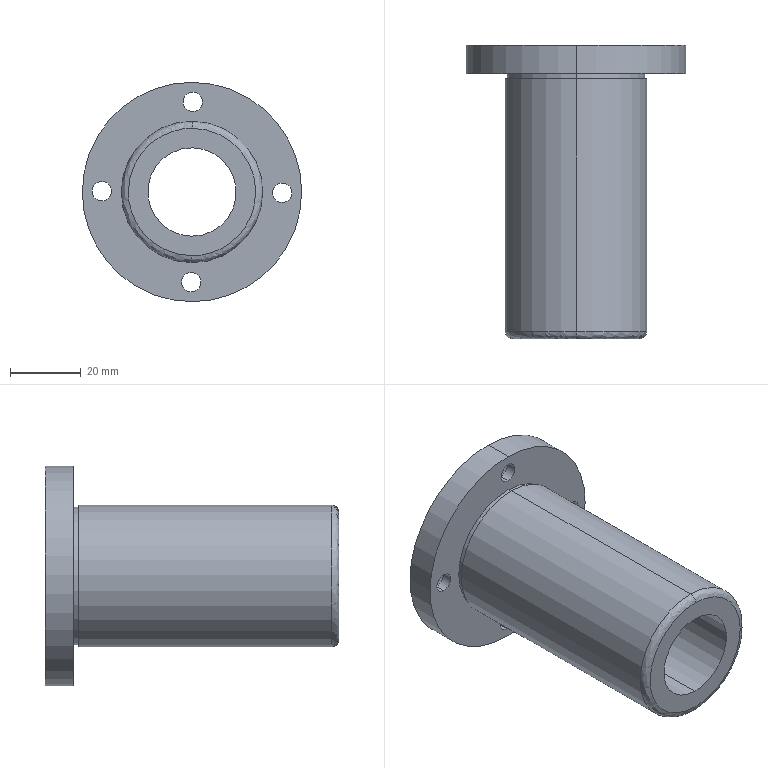Component | SolidWorks | LinearBearingMISUMILHFRD25-1 | 1 solid | 34 faces | box 62 x 83 x 62 mm | volume 75888 mm3 | cylinder 24 | plane 8 | spline 2 | commonest cylinder face diameters 5.5 x8 9 x8 40 x2 39 x2 25 x2 62 x2
STEP:
#1=CARTESIAN_POINT('',(5.125,-0.3937,7.677));
#2=VERTEX_POINT('',#1);
#3=CARTESIAN_POINT('',(5.111,-0.3937,6.102));
#4=VERTEX_POINT('',#3);
#5=CARTESIAN_POINT('',(5.118,-0.3937,6.89));
#6=DIRECTION('',(-0.,1.,-0.));
#7=DIRECTION('',(0.008424,0.,1.));
#8=AXIS2_PLACEMENT_3D('',#5,#6,#7);
#9=CIRCLE('',#8,0.7874);
#10=EDGE_CURVE('',#2,#4,#9,.T.);
#11=ORIENTED_EDGE('',*,*,#10,.F.);
#12=CARTESIAN_POINT('',(5.124,-0.4724,7.598));
#13=VERTEX_POINT('',#12);
#14=CARTESIAN_POINT('',(5.124,-0.3937,7.598));
#15=DIRECTION('',(1.,-0.,-0.008424));
#16=DIRECTION('',(0.008424,0.,1.));
#17=AXIS2_PLACEMENT_3D('',#14,#15,#16);
#18=CIRCLE('',#17,0.07874);
#19=EDGE_CURVE('',#2,#13,#18,.T.);
#20=ORIENTED_EDGE('',*,*,#19,.T.);
#21=CARTESIAN_POINT('',(5.112,-0.4724,6.181));
#22=VERTEX_POINT('',#21);
#23=CARTESIAN_POINT('',(5.124,-0.4724,7.598));
#24=CARTESIAN_POINT('',(6.541,-0.4724,7.586));
#25=CARTESIAN_POINT('',(6.529,-0.4724,6.169));
#26=CARTESIAN_POINT('',(5.112,-0.4724,6.181));
#27=(BOUNDED_CURVE()B_SPLINE_CURVE(3,(#23,#24,#25,#26),.UNSPECIFIED.,.F.,.T.)B_SPLINE_CURVE_WITH_KNOTS((4,4),(0.,1.),.UNSPECIFIED.)CURVE()GEOMETRIC_REPRESENTATION_ITEM()RATIONAL_B_SPLINE_CURVE((1.,0.3333,0.3333,1.))REPRESENTATION_ITEM(''));
#28=EDGE_CURVE('',#13,#22,#27,.T.);
#29=ORIENTED_EDGE('',*,*,#28,.T.);
#30=CARTESIAN_POINT('',(5.112,-0.3937,6.181));
#31=DIRECTION('',(-1.,0.,0.008424));
#32=DIRECTION('',(-0.008424,-0.,-1.));
#33=AXIS2_PLACEMENT_3D('',#30,#31,#32);
#34=CIRCLE('',#33,0.07874);
#35=EDGE_CURVE('',#4,#22,#34,.T.);
#36=ORIENTED_EDGE('',*,*,#35,.F.);
#37=EDGE_LOOP('',(#11,#20,#29,#36));
#38=FACE_OUTER_BOUND('',#37,.T.);
#39=CARTESIAN_POINT('',(5.125,-0.3937,7.677));
#40=CARTESIAN_POINT('',(6.699,-0.3937,7.664));
#41=CARTESIAN_POINT('',(6.686,-0.3937,6.089));
#42=CARTESIAN_POINT('',(5.111,-0.3937,6.102));
#43=CARTESIAN_POINT('',(5.125,-0.4398,7.677));
#44=CARTESIAN_POINT('',(6.699,-0.4398,7.664));
#45=CARTESIAN_POINT('',(6.686,-0.4398,6.089));
#46=CARTESIAN_POINT('',(5.111,-0.4398,6.102));
#47=CARTESIAN_POINT('',(5.124,-0.4724,7.645));
#48=CARTESIAN_POINT('',(6.634,-0.4724,7.632));
#49=CARTESIAN_POINT('',(6.621,-0.4724,6.122));
#50=CARTESIAN_POINT('',(5.112,-0.4724,6.135));
#51=CARTESIAN_POINT('',(5.124,-0.4724,7.598));
#52=CARTESIAN_POINT('',(6.541,-0.4724,7.586));
#53=CARTESIAN_POINT('',(6.529,-0.4724,6.169));
#54=CARTESIAN_POINT('',(5.112,-0.4724,6.181));
#55=(BOUNDED_SURFACE()B_SPLINE_SURFACE(3,3,((#39,#40,#41,#42),(#43,#44,#45,#46),(#47,#48,#49,#50),(#51,#52,#53,#54)),.UNSPECIFIED.,.F.,.F.,.T.)B_SPLINE_SURFACE_WITH_KNOTS((4,4),(4,4),(0.,1.),(0.,1.),.UNSPECIFIED.)GEOMETRIC_REPRESENTATION_ITEM()RATIONAL_B_SPLINE_SURFACE(((1.,0.3333,0.3333,1.),(0.8047,0.2682,0.2682,0.8047),(0.8047,0.2682,0.2682,0.8047),(1.,0.3333,0.3333,1.)))REPRESENTATION_ITEM('')SURFACE());
#56=ADVANCED_FACE('',(#38),#55,.T.);
#57=CARTESIAN_POINT('',(5.125,2.421,7.677));
#58=VERTEX_POINT('',#57);
#59=CARTESIAN_POINT('',(5.111,2.421,6.102));
#60=VERTEX_POINT('',#59);
#61=CARTESIAN_POINT('',(5.118,2.421,6.89));
#62=DIRECTION('',(0.,-1.,0.));
#63=DIRECTION('',(0.008424,0.,1.));
#64=AXIS2_PLACEMENT_3D('',#61,#62,#63);
#65=CIRCLE('',#64,0.7874);
#66=EDGE_CURVE('',#58,#60,#65,.T.);
#67=ORIENTED_EDGE('',*,*,#66,.T.);
#68=CARTESIAN_POINT('',(5.111,1.014,6.102));
#69=DIRECTION('',(0.,-1.,0.));
#70=VECTOR('',#69,39.37);
#71=LINE('',#68,#70);
#72=EDGE_CURVE('',#60,#4,#71,.T.);
#73=ORIENTED_EDGE('',*,*,#72,.T.);
#74=CARTESIAN_POINT('',(5.118,-0.3937,6.89));
#75=DIRECTION('',(-0.,1.,-0.));
#76=DIRECTION('',(0.008424,0.,1.));
#77=AXIS2_PLACEMENT_3D('',#74,#75,#76);
#78=CIRCLE('',#77,0.7874);
#79=EDGE_CURVE('',#4,#2,#78,.T.);
#80=ORIENTED_EDGE('',*,*,#79,.T.);
#81=CARTESIAN_POINT('',(5.125,1.014,7.677));
#82=DIRECTION('',(0.,-1.,0.));
#83=VECTOR('',#82,39.37);
#84=LINE('',#81,#83);
#85=EDGE_CURVE('',#58,#2,#84,.T.);
#86=ORIENTED_EDGE('',*,*,#85,.F.);
#87=EDGE_LOOP('',(#67,#73,#80,#86));
#88=FACE_OUTER_BOUND('',#87,.T.);
#89=CARTESIAN_POINT('',(5.118,1.014,6.89));
#90=DIRECTION('',(0.,-1.,0.));
#91=DIRECTION('',(0.008424,0.,1.));
#92=AXIS2_PLACEMENT_3D('',#89,#90,#91);
#93=CYLINDRICAL_SURFACE('',#92,0.7874);
#94=ADVANCED_FACE('',(#88),#93,.T.);
#95=CARTESIAN_POINT('',(5.125,2.48,7.657));
#96=VERTEX_POINT('',#95);
#97=CARTESIAN_POINT('',(5.112,2.48,6.122));
#98=VERTEX_POINT('',#97);
#99=CARTESIAN_POINT('',(5.118,2.48,6.89));
#100=DIRECTION('',(0.,-1.,0.));
#101=DIRECTION('',(0.008424,0.,1.));
#102=AXIS2_PLACEMENT_3D('',#99,#100,#101);
#103=CIRCLE('',#102,0.7677);
#104=EDGE_CURVE('',#96,#98,#103,.T.);
#105=ORIENTED_EDGE('',*,*,#104,.T.);
#106=CARTESIAN_POINT('',(5.112,2.421,6.122));
#107=VERTEX_POINT('',#106);
#108=CARTESIAN_POINT('',(5.112,2.451,6.122));
#109=DIRECTION('',(0.,-1.,0.));
#110=VECTOR('',#109,39.37);
#111=LINE('',#108,#110);
#112=EDGE_CURVE('',#98,#107,#111,.T.);
#113=ORIENTED_EDGE('',*,*,#112,.T.);
#114=CARTESIAN_POINT('',(5.125,2.421,7.657));
#115=VERTEX_POINT('',#114);
#116=CARTESIAN_POINT('',(5.118,2.421,6.89));
#117=DIRECTION('',(0.,-1.,0.));
#118=DIRECTION('',(0.008424,0.,1.));
#119=AXIS2_PLACEMENT_3D('',#116,#117,#118);
#120=CIRCLE('',#119,0.7677);
#121=EDGE_CURVE('',#115,#107,#120,.T.);
#122=ORIENTED_EDGE('',*,*,#121,.F.);
#123=CARTESIAN_POINT('',(5.125,2.451,7.657));
#124=DIRECTION('',(0.,-1.,0.));
#125=VECTOR('',#124,39.37);
#126=LINE('',#123,#125);
#127=EDGE_CURVE('',#96,#115,#126,.T.);
#128=ORIENTED_EDGE('',*,*,#127,.F.);
#129=EDGE_LOOP('',(#105,#113,#122,#128));
#130=FACE_OUTER_BOUND('',#129,.T.);
#131=CARTESIAN_POINT('',(5.118,2.451,6.89));
#132=DIRECTION('',(0.,-1.,0.));
#133=DIRECTION('',(0.008424,0.,1.));
#134=AXIS2_PLACEMENT_3D('',#131,#132,#133);
#135=CYLINDRICAL_SURFACE('',#134,0.7677);
#136=ADVANCED_FACE('',(#130),#135,.T.);
#137=CARTESIAN_POINT('',(5.114,2.795,6.398));
#138=VERTEX_POINT('',#137);
#139=CARTESIAN_POINT('',(5.122,2.795,7.382));
#140=VERTEX_POINT('',#139);
#141=CARTESIAN_POINT('',(5.118,2.795,6.89));
#142=DIRECTION('',(0.,-1.,0.));
#143=DIRECTION('',(0.008424,0.,1.));
#144=AXIS2_PLACEMENT_3D('',#141,#142,#143);
#145=CIRCLE('',#144,0.4921);
#146=EDGE_CURVE('',#138,#140,#145,.T.);
#147=ORIENTED_EDGE('',*,*,#146,.F.);
#148=CARTESIAN_POINT('',(5.114,-0.4724,6.398));
#149=VERTEX_POINT('',#148);
#150=CARTESIAN_POINT('',(5.114,1.161,6.398));
#151=DIRECTION('',(0.,-1.,0.));
#152=VECTOR('',#151,39.37);
#153=LINE('',#150,#152);
#154=EDGE_CURVE('',#138,#149,#153,.T.);
#155=ORIENTED_EDGE('',*,*,#154,.T.);
#156=CARTESIAN_POINT('',(5.122,-0.4724,7.382));
#157=VERTEX_POINT('',#156);
#158=CARTESIAN_POINT('',(5.118,-0.4724,6.89));
#159=DIRECTION('',(-0.,1.,-0.));
#160=DIRECTION('',(0.008424,0.,1.));
#161=AXIS2_PLACEMENT_3D('',#158,#159,#160);
#162=CIRCLE('',#161,0.4921);
#163=EDGE_CURVE('',#157,#149,#162,.T.);
#164=ORIENTED_EDGE('',*,*,#163,.F.);
#165=CARTESIAN_POINT('',(5.122,1.161,7.382));
#166=DIRECTION('',(0.,-1.,0.));
#167=VECTOR('',#166,39.37);
#168=LINE('',#165,#167);
#169=EDGE_CURVE('',#140,#157,#168,.T.);
#170=ORIENTED_EDGE('',*,*,#169,.F.);
#171=EDGE_LOOP('',(#147,#155,#164,#170));
#172=FACE_OUTER_BOUND('',#171,.T.);
#173=CARTESIAN_POINT('',(5.118,1.161,6.89));
#174=DIRECTION('',(0.,-1.,0.));
#175=DIRECTION('',(0.008424,0.,1.));
#176=AXIS2_PLACEMENT_3D('',#173,#174,#175);
#177=CYLINDRICAL_SURFACE('',#176,0.4921);
#178=ADVANCED_FACE('',(#172),#177,.F.);
#179=CARTESIAN_POINT('',(5.108,2.795,5.669));
#180=VERTEX_POINT('',#179);
#181=CARTESIAN_POINT('',(5.128,2.795,8.11));
#182=VERTEX_POINT('',#181);
#183=CARTESIAN_POINT('',(5.118,2.795,6.89));
#184=DIRECTION('',(-0.,1.,-0.));
#185=DIRECTION('',(0.008424,0.,1.));
#186=AXIS2_PLACEMENT_3D('',#183,#184,#185);
#187=CIRCLE('',#186,1.22);
#188=EDGE_CURVE('',#180,#182,#187,.T.);
#189=ORIENTED_EDGE('',*,*,#188,.F.);
#190=CARTESIAN_POINT('',(5.108,2.48,5.669));
#191=VERTEX_POINT('',#190);
#192=CARTESIAN_POINT('',(5.108,2.638,5.669));
#193=DIRECTION('',(0.,-1.,0.));
#194=VECTOR('',#193,39.37);
#195=LINE('',#192,#194);
#196=EDGE_CURVE('',#180,#191,#195,.T.);
#197=ORIENTED_EDGE('',*,*,#196,.T.);
#198=CARTESIAN_POINT('',(5.128,2.48,8.11));
#199=VERTEX_POINT('',#198);
#200=CARTESIAN_POINT('',(5.118,2.48,6.89));
#201=DIRECTION('',(0.,-1.,0.));
#202=DIRECTION('',(0.008424,0.,1.));
#203=AXIS2_PLACEMENT_3D('',#200,#201,#202);
#204=CIRCLE('',#203,1.22);
#205=EDGE_CURVE('',#199,#191,#204,.T.);
#206=ORIENTED_EDGE('',*,*,#205,.F.);
#207=CARTESIAN_POINT('',(5.128,2.638,8.11));
#208=DIRECTION('',(0.,-1.,0.));
#209=VECTOR('',#208,39.37);
#210=LINE('',#207,#209);
#211=EDGE_CURVE('',#182,#199,#210,.T.);
#212=ORIENTED_EDGE('',*,*,#211,.F.);
#213=EDGE_LOOP('',(#189,#197,#206,#212));
#214=FACE_OUTER_BOUND('',#213,.T.);
#215=CARTESIAN_POINT('',(5.118,2.638,6.89));
#216=DIRECTION('',(0.,-1.,0.));
#217=DIRECTION('',(0.008424,0.,1.));
#218=AXIS2_PLACEMENT_3D('',#215,#216,#217);
#219=CYLINDRICAL_SURFACE('',#218,1.22);
#220=ADVANCED_FACE('',(#214),#219,.T.);
#221=CARTESIAN_POINT('',(4.113,2.594,6.79));
#222=VERTEX_POINT('',#221);
#223=CARTESIAN_POINT('',(4.115,2.594,7.006));
#224=VERTEX_POINT('',#223);
#225=CARTESIAN_POINT('',(4.114,2.594,6.898));
#226=DIRECTION('',(0.,-1.,0.));
#227=DIRECTION('',(0.008424,0.,1.));
#228=AXIS2_PLACEMENT_3D('',#225,#226,#227);
#229=CIRCLE('',#228,0.1083);
#230=EDGE_CURVE('',#222,#224,#229,.T.);
#231=ORIENTED_EDGE('',*,*,#230,.F.);
#232=CARTESIAN_POINT('',(4.113,2.48,6.79));
#233=VERTEX_POINT('',#232);
#234=CARTESIAN_POINT('',(4.113,2.537,6.79));
#235=DIRECTION('',(0.,-1.,0.));
#236=VECTOR('',#235,39.37);
#237=LINE('',#234,#236);
#238=EDGE_CURVE('',#222,#233,#237,.T.);
#239=ORIENTED_EDGE('',*,*,#238,.T.);
#240=CARTESIAN_POINT('',(4.115,2.48,7.006));
#241=VERTEX_POINT('',#240);
#242=CARTESIAN_POINT('',(4.114,2.48,6.898));
#243=DIRECTION('',(-0.,1.,-0.));
#244=DIRECTION('',(0.008424,0.,1.));
#245=AXIS2_PLACEMENT_3D('',#242,#243,#244);
#246=CIRCLE('',#245,0.1083);
#247=EDGE_CURVE('',#241,#233,#246,.T.);
#248=ORIENTED_EDGE('',*,*,#247,.F.);
#249=CARTESIAN_POINT('',(4.115,2.537,7.006));
#250=DIRECTION('',(0.,-1.,0.));
#251=VECTOR('',#250,39.37);
#252=LINE('',#249,#251);
#253=EDGE_CURVE('',#224,#241,#252,.T.);
#254=ORIENTED_EDGE('',*,*,#253,.F.);
#255=EDGE_LOOP('',(#231,#239,#248,#254));
#256=FACE_OUTER_BOUND('',#255,.T.);
#257=CARTESIAN_POINT('',(4.114,2.537,6.898));
#258=DIRECTION('',(0.,-1.,0.));
#259=DIRECTION('',(0.008424,0.,1.));
#260=AXIS2_PLACEMENT_3D('',#257,#258,#259);
#261=CYLINDRICAL_SURFACE('',#260,0.1083);
#262=ADVANCED_FACE('',(#256),#261,.F.);
#263=CARTESIAN_POINT('',(5.126,2.594,7.785));
#264=VERTEX_POINT('',#263);
#265=CARTESIAN_POINT('',(5.127,2.594,8.002));
#266=VERTEX_POINT('',#265);
#267=CARTESIAN_POINT('',(5.127,2.594,7.894));
#268=DIRECTION('',(0.,-1.,0.));
#269=DIRECTION('',(0.008424,0.,1.));
#270=AXIS2_PLACEMENT_3D('',#267,#268,#269);
#271=CIRCLE('',#270,0.1083);
#272=EDGE_CURVE('',#264,#266,#271,.T.);
#273=ORIENTED_EDGE('',*,*,#272,.F.);
#274=CARTESIAN_POINT('',(5.126,2.48,7.785));
#275=VERTEX_POINT('',#274);
#276=CARTESIAN_POINT('',(5.126,2.537,7.785));
#277=DIRECTION('',(0.,-1.,0.));
#278=VECTOR('',#277,39.37);
#279=LINE('',#276,#278);
#280=EDGE_CURVE('',#264,#275,#279,.T.);
#281=ORIENTED_EDGE('',*,*,#280,.T.);
#282=CARTESIAN_POINT('',(5.127,2.48,8.002));
#283=VERTEX_POINT('',#282);
#284=CARTESIAN_POINT('',(5.127,2.48,7.894));
#285=DIRECTION('',(-0.,1.,-0.));
#286=DIRECTION('',(0.008424,0.,1.));
#287=AXIS2_PLACEMENT_3D('',#284,#285,#286);
#288=CIRCLE('',#287,0.1083);
#289=EDGE_CURVE('',#283,#275,#288,.T.);
#290=ORIENTED_EDGE('',*,*,#289,.F.);
#291=CARTESIAN_POINT('',(5.127,2.537,8.002));
#292=DIRECTION('',(0.,-1.,0.));
#293=VECTOR('',#292,39.37);
#294=LINE('',#291,#293);
#295=EDGE_CURVE('',#266,#283,#294,.T.);
#296=ORIENTED_EDGE('',*,*,#295,.F.);
#297=EDGE_LOOP('',(#273,#281,#290,#296));
#298=FACE_OUTER_BOUND('',#297,.T.);
#299=CARTESIAN_POINT('',(5.127,2.537,7.894));
#300=DIRECTION('',(0.,-1.,0.));
#301=DIRECTION('',(0.008424,0.,1.));
#302=AXIS2_PLACEMENT_3D('',#299,#300,#301);
#303=CYLINDRICAL_SURFACE('',#302,0.1083);
#304=ADVANCED_FACE('',(#298),#303,.F.);
#305=CARTESIAN_POINT('',(6.121,2.594,6.773));
#306=VERTEX_POINT('',#305);
#307=CARTESIAN_POINT('',(6.123,2.594,6.99));
#308=VERTEX_POINT('',#307);
#309=CARTESIAN_POINT('',(6.122,2.594,6.881));
#310=DIRECTION('',(0.,-1.,0.));
#311=DIRECTION('',(0.008424,0.,1.));
#312=AXIS2_PLACEMENT_3D('',#309,#310,#311);
#313=CIRCLE('',#312,0.1083);
#314=EDGE_CURVE('',#306,#308,#313,.T.);
#315=ORIENTED_EDGE('',*,*,#314,.F.);
#316=CARTESIAN_POINT('',(6.121,2.48,6.773));
#317=VERTEX_POINT('',#316);
#318=CARTESIAN_POINT('',(6.121,2.537,6.773));
#319=DIRECTION('',(0.,-1.,0.));
#320=VECTOR('',#319,39.37);
#321=LINE('',#318,#320);
#322=EDGE_CURVE('',#306,#317,#321,.T.);
#323=ORIENTED_EDGE('',*,*,#322,.T.);
#324=CARTESIAN_POINT('',(6.123,2.48,6.99));
#325=VERTEX_POINT('',#324);
#326=CARTESIAN_POINT('',(6.122,2.48,6.881));
#327=DIRECTION('',(-0.,1.,-0.));
#328=DIRECTION('',(0.008424,0.,1.));
#329=AXIS2_PLACEMENT_3D('',#326,#327,#328);
#330=CIRCLE('',#329,0.1083);
#331=EDGE_CURVE('',#325,#317,#330,.T.);
#332=ORIENTED_EDGE('',*,*,#331,.F.);
#333=CARTESIAN_POINT('',(6.123,2.537,6.99));
#334=DIRECTION('',(0.,-1.,0.));
#335=VECTOR('',#334,39.37);
#336=LINE('',#333,#335);
#337=EDGE_CURVE('',#308,#325,#336,.T.);
#338=ORIENTED_EDGE('',*,*,#337,.F.);
#339=EDGE_LOOP('',(#315,#323,#332,#338));
#340=FACE_OUTER_BOUND('',#339,.T.);
#341=CARTESIAN_POINT('',(6.122,2.537,6.881));
#342=DIRECTION('',(0.,-1.,0.));
#343=DIRECTION('',(0.008424,0.,1.));
#344=AXIS2_PLACEMENT_3D('',#341,#342,#343);
#345=CYLINDRICAL_SURFACE('',#344,0.1083);
#346=ADVANCED_FACE('',(#340),#345,.F.);
#347=CARTESIAN_POINT('',(5.109,2.594,5.778));
#348=VERTEX_POINT('',#347);
#349=CARTESIAN_POINT('',(5.111,2.594,5.994));
#350=VERTEX_POINT('',#349);
#351=CARTESIAN_POINT('',(5.11,2.594,5.886));
#352=DIRECTION('',(0.,-1.,0.));
#353=DIRECTION('',(0.008424,0.,1.));
#354=AXIS2_PLACEMENT_3D('',#351,#352,#353);
#355=CIRCLE('',#354,0.1083);
#356=EDGE_CURVE('',#348,#350,#355,.T.);
#357=ORIENTED_EDGE('',*,*,#356,.F.);
#358=CARTESIAN_POINT('',(5.109,2.48,5.778));
#359=VERTEX_POINT('',#358);
#360=CARTESIAN_POINT('',(5.109,2.537,5.778));
#361=DIRECTION('',(0.,-1.,0.));
#362=VECTOR('',#361,39.37);
#363=LINE('',#360,#362);
#364=EDGE_CURVE('',#348,#359,#363,.T.);
#365=ORIENTED_EDGE('',*,*,#364,.T.);
#366=CARTESIAN_POINT('',(5.111,2.48,5.994));
#367=VERTEX_POINT('',#366);
#368=CARTESIAN_POINT('',(5.11,2.48,5.886));
#369=DIRECTION('',(-0.,1.,-0.));
#370=DIRECTION('',(0.008424,0.,1.));
#371=AXIS2_PLACEMENT_3D('',#368,#369,#370);
#372=CIRCLE('',#371,0.1083);
#373=EDGE_CURVE('',#367,#359,#372,.T.);
#374=ORIENTED_EDGE('',*,*,#373,.F.);
#375=CARTESIAN_POINT('',(5.111,2.537,5.994));
#376=DIRECTION('',(0.,-1.,0.));
#377=VECTOR('',#376,39.37);
#378=LINE('',#375,#377);
#379=EDGE_CURVE('',#350,#367,#378,.T.);
#380=ORIENTED_EDGE('',*,*,#379,.F.);
#381=EDGE_LOOP('',(#357,#365,#374,#380));
#382=FACE_OUTER_BOUND('',#381,.T.);
#383=CARTESIAN_POINT('',(5.11,2.537,5.886));
#384=DIRECTION('',(0.,-1.,0.));
#385=DIRECTION('',(0.008424,0.,1.));
#386=AXIS2_PLACEMENT_3D('',#383,#384,#385);
#387=CYLINDRICAL_SURFACE('',#386,0.1083);
#388=ADVANCED_FACE('',(#382),#387,.F.);
#389=CARTESIAN_POINT('',(4.113,2.795,6.721));
#390=VERTEX_POINT('',#389);
#391=CARTESIAN_POINT('',(4.116,2.795,7.075));
#392=VERTEX_POINT('',#391);
#393=CARTESIAN_POINT('',(4.114,2.795,6.898));
#394=DIRECTION('',(0.,-1.,0.));
#395=DIRECTION('',(0.008424,0.,1.));
#396=AXIS2_PLACEMENT_3D('',#393,#394,#395);
#397=CIRCLE('',#396,0.1772);
#398=EDGE_CURVE('',#390,#392,#397,.T.);
#399=ORIENTED_EDGE('',*,*,#398,.F.);
#400=CARTESIAN_POINT('',(4.113,2.594,6.721));
#401=VERTEX_POINT('',#400);
#402=CARTESIAN_POINT('',(4.113,2.695,6.721));
#403=DIRECTION('',(0.,-1.,0.));
#404=VECTOR('',#403,39.37);
#405=LINE('',#402,#404);
#406=EDGE_CURVE('',#390,#401,#405,.T.);
#407=ORIENTED_EDGE('',*,*,#406,.T.);
#408=CARTESIAN_POINT('',(4.116,2.594,7.075));
#409=VERTEX_POINT('',#408);
#410=CARTESIAN_POINT('',(4.114,2.594,6.898));
#411=DIRECTION('',(-0.,1.,-0.));
#412=DIRECTION('',(0.008424,0.,1.));
#413=AXIS2_PLACEMENT_3D('',#410,#411,#412);
#414=CIRCLE('',#413,0.1772);
#415=EDGE_CURVE('',#409,#401,#414,.T.);
#416=ORIENTED_EDGE('',*,*,#415,.F.);
#417=CARTESIAN_POINT('',(4.116,2.695,7.075));
#418=DIRECTION('',(0.,-1.,0.));
#419=VECTOR('',#418,39.37);
#420=LINE('',#417,#419);
#421=EDGE_CURVE('',#392,#409,#420,.T.);
#422=ORIENTED_EDGE('',*,*,#421,.F.);
#423=EDGE_LOOP('',(#399,#407,#416,#422));
#424=FACE_OUTER_BOUND('',#423,.T.);
#425=CARTESIAN_POINT('',(4.114,2.695,6.898));
#426=DIRECTION('',(0.,-1.,0.));
#427=DIRECTION('',(0.008424,0.,1.));
#428=AXIS2_PLACEMENT_3D('',#425,#426,#427);
#429=CYLINDRICAL_SURFACE('',#428,0.1772);
#430=ADVANCED_FACE('',(#424),#429,.F.);
#431=CARTESIAN_POINT('',(5.125,2.795,7.717));
#432=VERTEX_POINT('',#431);
#433=CARTESIAN_POINT('',(5.128,2.795,8.071));
#434=VERTEX_POINT('',#433);
#435=CARTESIAN_POINT('',(5.127,2.795,7.894));
#436=DIRECTION('',(0.,-1.,0.));
#437=DIRECTION('',(0.008424,0.,1.));
#438=AXIS2_PLACEMENT_3D('',#435,#436,#437);
#439=CIRCLE('',#438,0.1772);
#440=EDGE_CURVE('',#432,#434,#439,.T.);
#441=ORIENTED_EDGE('',*,*,#440,.F.);
#442=CARTESIAN_POINT('',(5.125,2.594,7.717));
#443=VERTEX_POINT('',#442);
#444=CARTESIAN_POINT('',(5.125,2.695,7.717));
#445=DIRECTION('',(0.,-1.,0.));
#446=VECTOR('',#445,39.37);
#447=LINE('',#444,#446);
#448=EDGE_CURVE('',#432,#443,#447,.T.);
#449=ORIENTED_EDGE('',*,*,#448,.T.);
#450=CARTESIAN_POINT('',(5.128,2.594,8.071));
#451=VERTEX_POINT('',#450);
#452=CARTESIAN_POINT('',(5.127,2.594,7.894));
#453=DIRECTION('',(-0.,1.,-0.));
#454=DIRECTION('',(0.008424,0.,1.));
#455=AXIS2_PLACEMENT_3D('',#452,#453,#454);
#456=CIRCLE('',#455,0.1772);
#457=EDGE_CURVE('',#451,#443,#456,.T.);
#458=ORIENTED_EDGE('',*,*,#457,.F.);
#459=CARTESIAN_POINT('',(5.128,2.695,8.071));
#460=DIRECTION('',(0.,-1.,0.));
#461=VECTOR('',#460,39.37);
#462=LINE('',#459,#461);
#463=EDGE_CURVE('',#434,#451,#462,.T.);
#464=ORIENTED_EDGE('',*,*,#463,.F.);
#465=EDGE_LOOP('',(#441,#449,#458,#464));
#466=FACE_OUTER_BOUND('',#465,.T.);
#467=CARTESIAN_POINT('',(5.127,2.695,7.894));
#468=DIRECTION('',(0.,-1.,0.));
#469=DIRECTION('',(0.008424,0.,1.));
#470=AXIS2_PLACEMENT_3D('',#467,#468,#469);
#471=CYLINDRICAL_SURFACE('',#470,0.1772);
#472=ADVANCED_FACE('',(#466),#471,.F.);
#473=CARTESIAN_POINT('',(6.121,2.795,6.704));
#474=VERTEX_POINT('',#473);
#475=CARTESIAN_POINT('',(6.124,2.795,7.058));
#476=VERTEX_POINT('',#475);
#477=CARTESIAN_POINT('',(6.122,2.795,6.881));
#478=DIRECTION('',(0.,-1.,0.));
#479=DIRECTION('',(0.008424,0.,1.));
#480=AXIS2_PLACEMENT_3D('',#477,#478,#479);
#481=CIRCLE('',#480,0.1772);
#482=EDGE_CURVE('',#474,#476,#481,.T.);
#483=ORIENTED_EDGE('',*,*,#482,.F.);
#484=CARTESIAN_POINT('',(6.121,2.594,6.704));
#485=VERTEX_POINT('',#484);
#486=CARTESIAN_POINT('',(6.121,2.695,6.704));
#487=DIRECTION('',(0.,-1.,0.));
#488=VECTOR('',#487,39.37);
#489=LINE('',#486,#488);
#490=EDGE_CURVE('',#474,#485,#489,.T.);
#491=ORIENTED_EDGE('',*,*,#490,.T.);
#492=CARTESIAN_POINT('',(6.124,2.594,7.058));
#493=VERTEX_POINT('',#492);
#494=CARTESIAN_POINT('',(6.122,2.594,6.881));
#495=DIRECTION('',(-0.,1.,-0.));
#496=DIRECTION('',(0.008424,0.,1.));
#497=AXIS2_PLACEMENT_3D('',#494,#495,#496);
#498=CIRCLE('',#497,0.1772);
#499=EDGE_CURVE('',#493,#485,#498,.T.);
#500=ORIENTED_EDGE('',*,*,#499,.F.);
#501=CARTESIAN_POINT('',(6.124,2.695,7.058));
#502=DIRECTION('',(0.,-1.,0.));
#503=VECTOR('',#502,39.37);
#504=LINE('',#501,#503);
#505=EDGE_CURVE('',#476,#493,#504,.T.);
#506=ORIENTED_EDGE('',*,*,#505,.F.);
#507=EDGE_LOOP('',(#483,#491,#500,#506));
#508=FACE_OUTER_BOUND('',#507,.T.);
#509=CARTESIAN_POINT('',(6.122,2.695,6.881));
#510=DIRECTION('',(0.,-1.,0.));
#511=DIRECTION('',(0.008424,0.,1.));
#512=AXIS2_PLACEMENT_3D('',#509,#510,#511);
#513=CYLINDRICAL_SURFACE('',#512,0.1772);
#514=ADVANCED_FACE('',(#508),#513,.F.);
#515=CARTESIAN_POINT('',(5.108,2.795,5.709));
#516=VERTEX_POINT('',#515);
#517=CARTESIAN_POINT('',(5.111,2.795,6.063));
#518=VERTEX_POINT('',#517);
#519=CARTESIAN_POINT('',(5.11,2.795,5.886));
#520=DIRECTION('',(0.,-1.,0.));
#521=DIRECTION('',(0.008424,0.,1.));
#522=AXIS2_PLACEMENT_3D('',#519,#520,#521);
#523=CIRCLE('',#522,0.1772);
#524=EDGE_CURVE('',#516,#518,#523,.T.);
#525=ORIENTED_EDGE('',*,*,#524,.F.);
#526=CARTESIAN_POINT('',(5.108,2.594,5.709));
#527=VERTEX_POINT('',#526);
#528=CARTESIAN_POINT('',(5.108,2.695,5.709));
#529=DIRECTION('',(0.,-1.,0.));
#530=VECTOR('',#529,39.37);
#531=LINE('',#528,#530);
#532=EDGE_CURVE('',#516,#527,#531,.T.);
#533=ORIENTED_EDGE('',*,*,#532,.T.);
#534=CARTESIAN_POINT('',(5.111,2.594,6.063));
#535=VERTEX_POINT('',#534);
#536=CARTESIAN_POINT('',(5.11,2.594,5.886));
#537=DIRECTION('',(-0.,1.,-0.));
#538=DIRECTION('',(0.008424,0.,1.));
#539=AXIS2_PLACEMENT_3D('',#536,#537,#538);
#540=CIRCLE('',#539,0.1772);
#541=EDGE_CURVE('',#535,#527,#540,.T.);
#542=ORIENTED_EDGE('',*,*,#541,.F.);
#543=CARTESIAN_POINT('',(5.111,2.695,6.063));
#544=DIRECTION('',(0.,-1.,0.));
#545=VECTOR('',#544,39.37);
#546=LINE('',#543,#545);
#547=EDGE_CURVE('',#518,#535,#546,.T.);
#548=ORIENTED_EDGE('',*,*,#547,.F.);
#549=EDGE_LOOP('',(#525,#533,#542,#548));
#550=FACE_OUTER_BOUND('',#549,.T.);
#551=CARTESIAN_POINT('',(5.11,2.695,5.886));
#552=DIRECTION('',(0.,-1.,0.));
#553=DIRECTION('',(0.008424,0.,1.));
#554=AXIS2_PLACEMENT_3D('',#551,#552,#553);
#555=CYLINDRICAL_SURFACE('',#554,0.1772);
#556=ADVANCED_FACE('',(#550),#555,.F.);
#557=ORIENTED_EDGE('',*,*,#72,.F.);
#558=CARTESIAN_POINT('',(5.118,2.421,6.89));
#559=DIRECTION('',(0.,-1.,0.));
#560=DIRECTION('',(0.008424,0.,1.));
#561=AXIS2_PLACEMENT_3D('',#558,#559,#560);
#562=CIRCLE('',#561,0.7874);
#563=EDGE_CURVE('',#60,#58,#562,.T.);
#564=ORIENTED_EDGE('',*,*,#563,.T.);
#565=ORIENTED_EDGE('',*,*,#85,.T.);
#566=ORIENTED_EDGE('',*,*,#10,.T.);
#567=EDGE_LOOP('',(#557,#564,#565,#566));
#568=FACE_OUTER_BOUND('',#567,.T.);
#569=CARTESIAN_POINT('',(5.118,1.014,6.89));
#570=DIRECTION('',(0.,-1.,0.));
#571=DIRECTION('',(0.008424,0.,1.));
#572=AXIS2_PLACEMENT_3D('',#569,#570,#571);
#573=CYLINDRICAL_SURFACE('',#572,0.7874);
#574=ADVANCED_FACE('',(#568),#573,.T.);
#575=ORIENTED_EDGE('',*,*,#19,.F.);
#576=ORIENTED_EDGE('',*,*,#79,.F.);
#577=ORIENTED_EDGE('',*,*,#35,.T.);
#578=CARTESIAN_POINT('',(4.409,-0.4724,6.896));
#579=VERTEX_POINT('',#578);
#580=CARTESIAN_POINT('',(5.112,-0.4724,6.181));
#581=CARTESIAN_POINT('',(4.697,-0.4724,6.185));
#582=CARTESIAN_POINT('',(4.406,-0.4724,6.481));
#583=CARTESIAN_POINT('',(4.409,-0.4724,6.896));
#584=(BOUNDED_CURVE()B_SPLINE_CURVE(3,(#580,#581,#582,#583),.UNSPECIFIED.,.F.,.T.)B_SPLINE_CURVE_WITH_KNOTS((4,4),(0.,1.),.UNSPECIFIED.)CURVE()GEOMETRIC_REPRESENTATION_ITEM()RATIONAL_B_SPLINE_CURVE((1.,0.8047,0.8047,1.))REPRESENTATION_ITEM(''));
#585=EDGE_CURVE('',#22,#579,#584,.T.);
#586=ORIENTED_EDGE('',*,*,#585,.T.);
#587=CARTESIAN_POINT('',(4.409,-0.4724,6.896));
#588=CARTESIAN_POINT('',(4.413,-0.4724,7.311));
#589=CARTESIAN_POINT('',(4.709,-0.4724,7.602));
#590=CARTESIAN_POINT('',(5.124,-0.4724,7.598));
#591=(BOUNDED_CURVE()B_SPLINE_CURVE(3,(#587,#588,#589,#590),.UNSPECIFIED.,.F.,.T.)B_SPLINE_CURVE_WITH_KNOTS((4,4),(0.,1.),.UNSPECIFIED.)CURVE()GEOMETRIC_REPRESENTATION_ITEM()RATIONAL_B_SPLINE_CURVE((1.,0.8047,0.8047,1.))REPRESENTATION_ITEM(''));
#592=EDGE_CURVE('',#579,#13,#591,.T.);
#593=ORIENTED_EDGE('',*,*,#592,.T.);
#594=EDGE_LOOP('',(#575,#576,#577,#586,#593));
#595=FACE_OUTER_BOUND('',#594,.T.);
#596=CARTESIAN_POINT('',(5.111,-0.3937,6.102));
#597=CARTESIAN_POINT('',(3.537,-0.3937,6.116));
#598=CARTESIAN_POINT('',(3.55,-0.3937,7.69));
#599=CARTESIAN_POINT('',(5.125,-0.3937,7.677));
#600=CARTESIAN_POINT('',(5.111,-0.4398,6.102));
#601=CARTESIAN_POINT('',(3.537,-0.4398,6.116));
#602=CARTESIAN_POINT('',(3.55,-0.4398,7.69));
#603=CARTESIAN_POINT('',(5.125,-0.4398,7.677));
#604=CARTESIAN_POINT('',(5.112,-0.4724,6.135));
#605=CARTESIAN_POINT('',(3.602,-0.4724,6.148));
#606=CARTESIAN_POINT('',(3.615,-0.4724,7.657));
#607=CARTESIAN_POINT('',(5.124,-0.4724,7.645));
#608=CARTESIAN_POINT('',(5.112,-0.4724,6.181));
#609=CARTESIAN_POINT('',(3.695,-0.4724,6.193));
#610=CARTESIAN_POINT('',(3.707,-0.4724,7.61));
#611=CARTESIAN_POINT('',(5.124,-0.4724,7.598));
#612=(BOUNDED_SURFACE()B_SPLINE_SURFACE(3,3,((#596,#597,#598,#599),(#600,#601,#602,#603),(#604,#605,#606,#607),(#608,#609,#610,#611)),.UNSPECIFIED.,.F.,.F.,.T.)B_SPLINE_SURFACE_WITH_KNOTS((4,4),(4,4),(0.,1.),(0.,1.),.UNSPECIFIED.)GEOMETRIC_REPRESENTATION_ITEM()RATIONAL_B_SPLINE_SURFACE(((1.,0.3333,0.3333,1.),(0.8047,0.2682,0.2682,0.8047),(0.8047,0.2682,0.2682,0.8047),(1.,0.3333,0.3333,1.)))REPRESENTATION_ITEM('')SURFACE());
#613=ADVANCED_FACE('',(#595),#612,.T.);
#614=ORIENTED_EDGE('',*,*,#66,.F.);
#615=ORIENTED_EDGE('',*,*,#563,.F.);
#616=EDGE_LOOP('',(#614,#615));
#617=FACE_OUTER_BOUND('',#616,.T.);
#618=ORIENTED_EDGE('',*,*,#121,.T.);
#619=CARTESIAN_POINT('',(5.118,2.421,6.89));
#620=DIRECTION('',(0.,-1.,0.));
#621=DIRECTION('',(0.008424,0.,1.));
#622=AXIS2_PLACEMENT_3D('',#619,#620,#621);
#623=CIRCLE('',#622,0.7677);
#624=EDGE_CURVE('',#107,#115,#623,.T.);
#625=ORIENTED_EDGE('',*,*,#624,.T.);
#626=EDGE_LOOP('',(#618,#625));
#627=FACE_BOUND('',#626,.T.);
#628=CARTESIAN_POINT('',(4.341,2.421,6.896));
#629=DIRECTION('',(-0.,1.,-0.));
#630=DIRECTION('',(-0.008424,-0.,-1.));
#631=AXIS2_PLACEMENT_3D('',#628,#629,#630);
#632=PLANE('',#631);
#633=ADVANCED_FACE('',(#617,#627),#632,.T.);
#634=ORIENTED_EDGE('',*,*,#163,.T.);
#635=CARTESIAN_POINT('',(5.118,-0.4724,6.89));
#636=DIRECTION('',(-0.,1.,-0.));
#637=DIRECTION('',(0.008424,0.,1.));
#638=AXIS2_PLACEMENT_3D('',#635,#636,#637);
#639=CIRCLE('',#638,0.4921);
#640=EDGE_CURVE('',#149,#157,#639,.T.);
#641=ORIENTED_EDGE('',*,*,#640,.T.);
#642=EDGE_LOOP('',(#634,#641));
#643=FACE_BOUND('',#642,.T.);
#644=ORIENTED_EDGE('',*,*,#585,.F.);
#645=ORIENTED_EDGE('',*,*,#28,.F.);
#646=ORIENTED_EDGE('',*,*,#592,.F.);
#647=EDGE_LOOP('',(#644,#645,#646));
#648=FACE_OUTER_BOUND('',#647,.T.);
#649=CARTESIAN_POINT('',(4.518,-0.4724,6.895));
#650=DIRECTION('',(0.,-1.,0.));
#651=DIRECTION('',(0.008424,0.,1.));
#652=AXIS2_PLACEMENT_3D('',#649,#650,#651);
#653=PLANE('',#652);
#654=ADVANCED_FACE('',(#643,#648),#653,.T.);
#655=ORIENTED_EDGE('',*,*,#112,.F.);
#656=CARTESIAN_POINT('',(5.118,2.48,6.89));
#657=DIRECTION('',(0.,-1.,0.));
#658=DIRECTION('',(0.008424,0.,1.));
#659=AXIS2_PLACEMENT_3D('',#656,#657,#658);
#660=CIRCLE('',#659,0.7677);
#661=EDGE_CURVE('',#98,#96,#660,.T.);
#662=ORIENTED_EDGE('',*,*,#661,.T.);
#663=ORIENTED_EDGE('',*,*,#127,.T.);
#664=ORIENTED_EDGE('',*,*,#624,.F.);
#665=EDGE_LOOP('',(#655,#662,#663,#664));
#666=FACE_OUTER_BOUND('',#665,.T.);
#667=CARTESIAN_POINT('',(5.118,2.451,6.89));
#668=DIRECTION('',(0.,-1.,0.));
#669=DIRECTION('',(0.008424,0.,1.));
#670=AXIS2_PLACEMENT_3D('',#667,#668,#669);
#671=CYLINDRICAL_SURFACE('',#670,0.7677);
#672=ADVANCED_FACE('',(#666),#671,.T.);
#673=ORIENTED_EDGE('',*,*,#154,.F.);
#674=CARTESIAN_POINT('',(5.118,2.795,6.89));
#675=DIRECTION('',(0.,-1.,0.));
#676=DIRECTION('',(0.008424,0.,1.));
#677=AXIS2_PLACEMENT_3D('',#674,#675,#676);
#678=CIRCLE('',#677,0.4921);
#679=EDGE_CURVE('',#140,#138,#678,.T.);
#680=ORIENTED_EDGE('',*,*,#679,.F.);
#681=ORIENTED_EDGE('',*,*,#169,.T.);
#682=ORIENTED_EDGE('',*,*,#640,.F.);
#683=EDGE_LOOP('',(#673,#680,#681,#682));
#684=FACE_OUTER_BOUND('',#683,.T.);
#685=CARTESIAN_POINT('',(5.118,1.161,6.89));
#686=DIRECTION('',(0.,-1.,0.));
#687=DIRECTION('',(0.008424,0.,1.));
#688=AXIS2_PLACEMENT_3D('',#685,#686,#687);
#689=CYLINDRICAL_SURFACE('',#688,0.4921);
#690=ADVANCED_FACE('',(#684),#689,.F.);
#691=ORIENTED_EDGE('',*,*,#104,.F.);
#692=ORIENTED_EDGE('',*,*,#661,.F.);
#693=EDGE_LOOP('',(#691,#692));
#694=FACE_BOUND('',#693,.T.);
#695=ORIENTED_EDGE('',*,*,#205,.T.);
#696=CARTESIAN_POINT('',(5.118,2.48,6.89));
#697=DIRECTION('',(0.,-1.,0.));
#698=DIRECTION('',(0.008424,0.,1.));
#699=AXIS2_PLACEMENT_3D('',#696,#697,#698);
#700=CIRCLE('',#699,1.22);
#701=EDGE_CURVE('',#191,#199,#700,.T.);
#702=ORIENTED_EDGE('',*,*,#701,.T.);
#703=EDGE_LOOP('',(#695,#702));
#704=FACE_OUTER_BOUND('',#703,.T.);
#705=ORIENTED_EDGE('',*,*,#247,.T.);
#706=CARTESIAN_POINT('',(4.114,2.48,6.898));
#707=DIRECTION('',(-0.,1.,-0.));
#708=DIRECTION('',(0.008424,0.,1.));
#709=AXIS2_PLACEMENT_3D('',#706,#707,#708);
#710=CIRCLE('',#709,0.1083);
#711=EDGE_CURVE('',#233,#241,#710,.T.);
#712=ORIENTED_EDGE('',*,*,#711,.T.);
#713=EDGE_LOOP('',(#705,#712));
#714=FACE_BOUND('',#713,.T.);
#715=ORIENTED_EDGE('',*,*,#289,.T.);
#716=CARTESIAN_POINT('',(5.127,2.48,7.894));
#717=DIRECTION('',(-0.,1.,-0.));
#718=DIRECTION('',(0.008424,0.,1.));
#719=AXIS2_PLACEMENT_3D('',#716,#717,#718);
#720=CIRCLE('',#719,0.1083);
#721=EDGE_CURVE('',#275,#283,#720,.T.);
#722=ORIENTED_EDGE('',*,*,#721,.T.);
#723=EDGE_LOOP('',(#715,#722));
#724=FACE_BOUND('',#723,.T.);
#725=ORIENTED_EDGE('',*,*,#331,.T.);
#726=CARTESIAN_POINT('',(6.122,2.48,6.881));
#727=DIRECTION('',(-0.,1.,-0.));
#728=DIRECTION('',(0.008424,0.,1.));
#729=AXIS2_PLACEMENT_3D('',#726,#727,#728);
#730=CIRCLE('',#729,0.1083);
#731=EDGE_CURVE('',#317,#325,#730,.T.);
#732=ORIENTED_EDGE('',*,*,#731,.T.);
#733=EDGE_LOOP('',(#725,#732));
#734=FACE_BOUND('',#733,.T.);
#735=ORIENTED_EDGE('',*,*,#373,.T.);
#736=CARTESIAN_POINT('',(5.11,2.48,5.886));
#737=DIRECTION('',(-0.,1.,-0.));
#738=DIRECTION('',(0.008424,0.,1.));
#739=AXIS2_PLACEMENT_3D('',#736,#737,#738);
#740=CIRCLE('',#739,0.1083);
#741=EDGE_CURVE('',#359,#367,#740,.T.);
#742=ORIENTED_EDGE('',*,*,#741,.T.);
#743=EDGE_LOOP('',(#735,#742));
#744=FACE_BOUND('',#743,.T.);
#745=CARTESIAN_POINT('',(4.124,2.48,6.898));
#746=DIRECTION('',(0.,-1.,0.));
#747=DIRECTION('',(0.008424,0.,1.));
#748=AXIS2_PLACEMENT_3D('',#745,#746,#747);
#749=PLANE('',#748);
#750=ADVANCED_FACE('',(#694,#704,#714,#724,#734,#744),#749,.T.);
#751=CARTESIAN_POINT('',(5.118,2.795,6.89));
#752=DIRECTION('',(-0.,1.,-0.));
#753=DIRECTION('',(0.008424,0.,1.));
#754=AXIS2_PLACEMENT_3D('',#751,#752,#753);
#755=CIRCLE('',#754,1.22);
#756=EDGE_CURVE('',#182,#180,#755,.T.);
#757=ORIENTED_EDGE('',*,*,#756,.T.);
#758=ORIENTED_EDGE('',*,*,#188,.T.);
#759=EDGE_LOOP('',(#757,#758));
#760=FACE_OUTER_BOUND('',#759,.T.);
#761=ORIENTED_EDGE('',*,*,#679,.T.);
#762=ORIENTED_EDGE('',*,*,#146,.T.);
#763=EDGE_LOOP('',(#761,#762));
#764=FACE_BOUND('',#763,.T.);
#765=CARTESIAN_POINT('',(4.114,2.795,6.898));
#766=DIRECTION('',(0.,-1.,0.));
#767=DIRECTION('',(0.008424,0.,1.));
#768=AXIS2_PLACEMENT_3D('',#765,#766,#767);
#769=CIRCLE('',#768,0.1772);
#770=EDGE_CURVE('',#392,#390,#769,.T.);
#771=ORIENTED_EDGE('',*,*,#770,.T.);
#772=ORIENTED_EDGE('',*,*,#398,.T.);
#773=EDGE_LOOP('',(#771,#772));
#774=FACE_BOUND('',#773,.T.);
#775=CARTESIAN_POINT('',(5.127,2.795,7.894));
#776=DIRECTION('',(0.,-1.,0.));
#777=DIRECTION('',(0.008424,0.,1.));
#778=AXIS2_PLACEMENT_3D('',#775,#776,#777);
#779=CIRCLE('',#778,0.1772);
#780=EDGE_CURVE('',#434,#432,#779,.T.);
#781=ORIENTED_EDGE('',*,*,#780,.T.);
#782=ORIENTED_EDGE('',*,*,#440,.T.);
#783=EDGE_LOOP('',(#781,#782));
#784=FACE_BOUND('',#783,.T.);
#785=CARTESIAN_POINT('',(6.122,2.795,6.881));
#786=DIRECTION('',(0.,-1.,0.));
#787=DIRECTION('',(0.008424,0.,1.));
#788=AXIS2_PLACEMENT_3D('',#785,#786,#787);
#789=CIRCLE('',#788,0.1772);
#790=EDGE_CURVE('',#476,#474,#789,.T.);
#791=ORIENTED_EDGE('',*,*,#790,.T.);
#792=ORIENTED_EDGE('',*,*,#482,.T.);
#793=EDGE_LOOP('',(#791,#792));
#794=FACE_BOUND('',#793,.T.);
#795=CARTESIAN_POINT('',(5.11,2.795,5.886));
#796=DIRECTION('',(0.,-1.,0.));
#797=DIRECTION('',(0.008424,0.,1.));
#798=AXIS2_PLACEMENT_3D('',#795,#796,#797);
#799=CIRCLE('',#798,0.1772);
#800=EDGE_CURVE('',#518,#516,#799,.T.);
#801=ORIENTED_EDGE('',*,*,#800,.T.);
#802=ORIENTED_EDGE('',*,*,#524,.T.);
#803=EDGE_LOOP('',(#801,#802));
#804=FACE_BOUND('',#803,.T.);
#805=CARTESIAN_POINT('',(4.262,2.795,6.897));
#806=DIRECTION('',(-0.,1.,-0.));
#807=DIRECTION('',(-0.008424,-0.,-1.));
#808=AXIS2_PLACEMENT_3D('',#805,#806,#807);
#809=PLANE('',#808);
#810=ADVANCED_FACE('',(#760,#764,#774,#784,#794,#804),#809,.T.);
#811=ORIENTED_EDGE('',*,*,#196,.F.);
#812=ORIENTED_EDGE('',*,*,#756,.F.);
#813=ORIENTED_EDGE('',*,*,#211,.T.);
#814=ORIENTED_EDGE('',*,*,#701,.F.);
#815=EDGE_LOOP('',(#811,#812,#813,#814));
#816=FACE_OUTER_BOUND('',#815,.T.);
#817=CARTESIAN_POINT('',(5.118,2.638,6.89));
#818=DIRECTION('',(0.,-1.,0.));
#819=DIRECTION('',(0.008424,0.,1.));
#820=AXIS2_PLACEMENT_3D('',#817,#818,#819);
#821=CYLINDRICAL_SURFACE('',#820,1.22);
#822=ADVANCED_FACE('',(#816),#821,.T.);
#823=ORIENTED_EDGE('',*,*,#238,.F.);
#824=CARTESIAN_POINT('',(4.114,2.594,6.898));
#825=DIRECTION('',(0.,-1.,0.));
#826=DIRECTION('',(0.008424,0.,1.));
#827=AXIS2_PLACEMENT_3D('',#824,#825,#826);
#828=CIRCLE('',#827,0.1083);
#829=EDGE_CURVE('',#224,#222,#828,.T.);
#830=ORIENTED_EDGE('',*,*,#829,.F.);
#831=ORIENTED_EDGE('',*,*,#253,.T.);
#832=ORIENTED_EDGE('',*,*,#711,.F.);
#833=EDGE_LOOP('',(#823,#830,#831,#832));
#834=FACE_OUTER_BOUND('',#833,.T.);
#835=CARTESIAN_POINT('',(4.114,2.537,6.898));
#836=DIRECTION('',(0.,-1.,0.));
#837=DIRECTION('',(0.008424,0.,1.));
#838=AXIS2_PLACEMENT_3D('',#835,#836,#837);
#839=CYLINDRICAL_SURFACE('',#838,0.1083);
#840=ADVANCED_FACE('',(#834),#839,.F.);
#841=ORIENTED_EDGE('',*,*,#280,.F.);
#842=CARTESIAN_POINT('',(5.127,2.594,7.894));
#843=DIRECTION('',(0.,-1.,0.));
#844=DIRECTION('',(0.008424,0.,1.));
#845=AXIS2_PLACEMENT_3D('',#842,#843,#844);
#846=CIRCLE('',#845,0.1083);
#847=EDGE_CURVE('',#266,#264,#846,.T.);
#848=ORIENTED_EDGE('',*,*,#847,.F.);
#849=ORIENTED_EDGE('',*,*,#295,.T.);
#850=ORIENTED_EDGE('',*,*,#721,.F.);
#851=EDGE_LOOP('',(#841,#848,#849,#850));
#852=FACE_OUTER_BOUND('',#851,.T.);
#853=CARTESIAN_POINT('',(5.127,2.537,7.894));
#854=DIRECTION('',(0.,-1.,0.));
#855=DIRECTION('',(0.008424,0.,1.));
#856=AXIS2_PLACEMENT_3D('',#853,#854,#855);
#857=CYLINDRICAL_SURFACE('',#856,0.1083);
#858=ADVANCED_FACE('',(#852),#857,.F.);
#859=ORIENTED_EDGE('',*,*,#322,.F.);
#860=CARTESIAN_POINT('',(6.122,2.594,6.881));
#861=DIRECTION('',(0.,-1.,0.));
#862=DIRECTION('',(0.008424,0.,1.));
#863=AXIS2_PLACEMENT_3D('',#860,#861,#862);
#864=CIRCLE('',#863,0.1083);
#865=EDGE_CURVE('',#308,#306,#864,.T.);
#866=ORIENTED_EDGE('',*,*,#865,.F.);
#867=ORIENTED_EDGE('',*,*,#337,.T.);
#868=ORIENTED_EDGE('',*,*,#731,.F.);
#869=EDGE_LOOP('',(#859,#866,#867,#868));
#870=FACE_OUTER_BOUND('',#869,.T.);
#871=CARTESIAN_POINT('',(6.122,2.537,6.881));
#872=DIRECTION('',(0.,-1.,0.));
#873=DIRECTION('',(0.008424,0.,1.));
#874=AXIS2_PLACEMENT_3D('',#871,#872,#873);
#875=CYLINDRICAL_SURFACE('',#874,0.1083);
#876=ADVANCED_FACE('',(#870),#875,.F.);
#877=ORIENTED_EDGE('',*,*,#364,.F.);
#878=CARTESIAN_POINT('',(5.11,2.594,5.886));
#879=DIRECTION('',(0.,-1.,0.));
#880=DIRECTION('',(0.008424,0.,1.));
#881=AXIS2_PLACEMENT_3D('',#878,#879,#880);
#882=CIRCLE('',#881,0.1083);
#883=EDGE_CURVE('',#350,#348,#882,.T.);
#884=ORIENTED_EDGE('',*,*,#883,.F.);
#885=ORIENTED_EDGE('',*,*,#379,.T.);
#886=ORIENTED_EDGE('',*,*,#741,.F.);
#887=EDGE_LOOP('',(#877,#884,#885,#886));
#888=FACE_OUTER_BOUND('',#887,.T.);
#889=CARTESIAN_POINT('',(5.11,2.537,5.886));
#890=DIRECTION('',(0.,-1.,0.));
#891=DIRECTION('',(0.008424,0.,1.));
#892=AXIS2_PLACEMENT_3D('',#889,#890,#891);
#893=CYLINDRICAL_SURFACE('',#892,0.1083);
#894=ADVANCED_FACE('',(#888),#893,.F.);
#895=ORIENTED_EDGE('',*,*,#406,.F.);
#896=ORIENTED_EDGE('',*,*,#770,.F.);
#897=ORIENTED_EDGE('',*,*,#421,.T.);
#898=CARTESIAN_POINT('',(4.114,2.594,6.898));
#899=DIRECTION('',(-0.,1.,-0.));
#900=DIRECTION('',(0.008424,0.,1.));
#901=AXIS2_PLACEMENT_3D('',#898,#899,#900);
#902=CIRCLE('',#901,0.1772);
#903=EDGE_CURVE('',#401,#409,#902,.T.);
#904=ORIENTED_EDGE('',*,*,#903,.F.);
#905=EDGE_LOOP('',(#895,#896,#897,#904));
#906=FACE_OUTER_BOUND('',#905,.T.);
#907=CARTESIAN_POINT('',(4.114,2.695,6.898));
#908=DIRECTION('',(0.,-1.,0.));
#909=DIRECTION('',(0.008424,0.,1.));
#910=AXIS2_PLACEMENT_3D('',#907,#908,#909);
#911=CYLINDRICAL_SURFACE('',#910,0.1772);
#912=ADVANCED_FACE('',(#906),#911,.F.);
#913=ORIENTED_EDGE('',*,*,#448,.F.);
#914=ORIENTED_EDGE('',*,*,#780,.F.);
#915=ORIENTED_EDGE('',*,*,#463,.T.);
#916=CARTESIAN_POINT('',(5.127,2.594,7.894));
#917=DIRECTION('',(-0.,1.,-0.));
#918=DIRECTION('',(0.008424,0.,1.));
#919=AXIS2_PLACEMENT_3D('',#916,#917,#918);
#920=CIRCLE('',#919,0.1772);
#921=EDGE_CURVE('',#443,#451,#920,.T.);
#922=ORIENTED_EDGE('',*,*,#921,.F.);
#923=EDGE_LOOP('',(#913,#914,#915,#922));
#924=FACE_OUTER_BOUND('',#923,.T.);
#925=CARTESIAN_POINT('',(5.127,2.695,7.894));
#926=DIRECTION('',(0.,-1.,0.));
#927=DIRECTION('',(0.008424,0.,1.));
#928=AXIS2_PLACEMENT_3D('',#925,#926,#927);
#929=CYLINDRICAL_SURFACE('',#928,0.1772);
#930=ADVANCED_FACE('',(#924),#929,.F.);
#931=ORIENTED_EDGE('',*,*,#490,.F.);
#932=ORIENTED_EDGE('',*,*,#790,.F.);
#933=ORIENTED_EDGE('',*,*,#505,.T.);
#934=CARTESIAN_POINT('',(6.122,2.594,6.881));
#935=DIRECTION('',(-0.,1.,-0.));
#936=DIRECTION('',(0.008424,0.,1.));
#937=AXIS2_PLACEMENT_3D('',#934,#935,#936);
#938=CIRCLE('',#937,0.1772);
#939=EDGE_CURVE('',#485,#493,#938,.T.);
#940=ORIENTED_EDGE('',*,*,#939,.F.);
#941=EDGE_LOOP('',(#931,#932,#933,#940));
#942=FACE_OUTER_BOUND('',#941,.T.);
#943=CARTESIAN_POINT('',(6.122,2.695,6.881));
#944=DIRECTION('',(0.,-1.,0.));
#945=DIRECTION('',(0.008424,0.,1.));
#946=AXIS2_PLACEMENT_3D('',#943,#944,#945);
#947=CYLINDRICAL_SURFACE('',#946,0.1772);
#948=ADVANCED_FACE('',(#942),#947,.F.);
#949=ORIENTED_EDGE('',*,*,#532,.F.);
#950=ORIENTED_EDGE('',*,*,#800,.F.);
#951=ORIENTED_EDGE('',*,*,#547,.T.);
#952=CARTESIAN_POINT('',(5.11,2.594,5.886));
#953=DIRECTION('',(-0.,1.,-0.));
#954=DIRECTION('',(0.008424,0.,1.));
#955=AXIS2_PLACEMENT_3D('',#952,#953,#954);
#956=CIRCLE('',#955,0.1772);
#957=EDGE_CURVE('',#527,#535,#956,.T.);
#958=ORIENTED_EDGE('',*,*,#957,.F.);
#959=EDGE_LOOP('',(#949,#950,#951,#958));
#960=FACE_OUTER_BOUND('',#959,.T.);
#961=CARTESIAN_POINT('',(5.11,2.695,5.886));
#962=DIRECTION('',(0.,-1.,0.));
#963=DIRECTION('',(0.008424,0.,1.));
#964=AXIS2_PLACEMENT_3D('',#961,#962,#963);
#965=CYLINDRICAL_SURFACE('',#964,0.1772);
#966=ADVANCED_FACE('',(#960),#965,.F.);
#967=ORIENTED_EDGE('',*,*,#829,.T.);
#968=ORIENTED_EDGE('',*,*,#230,.T.);
#969=EDGE_LOOP('',(#967,#968));
#970=FACE_BOUND('',#969,.T.);
#971=ORIENTED_EDGE('',*,*,#415,.T.);
#972=ORIENTED_EDGE('',*,*,#903,.T.);
#973=EDGE_LOOP('',(#971,#972));
#974=FACE_OUTER_BOUND('',#973,.T.);
#975=CARTESIAN_POINT('',(3.971,2.594,6.899));
#976=DIRECTION('',(0.,-1.,0.));
#977=DIRECTION('',(0.008424,0.,1.));
#978=AXIS2_PLACEMENT_3D('',#975,#976,#977);
#979=PLANE('',#978);
#980=ADVANCED_FACE('',(#970,#974),#979,.F.);
#981=ORIENTED_EDGE('',*,*,#847,.T.);
#982=ORIENTED_EDGE('',*,*,#272,.T.);
#983=EDGE_LOOP('',(#981,#982));
#984=FACE_BOUND('',#983,.T.);
#985=ORIENTED_EDGE('',*,*,#457,.T.);
#986=ORIENTED_EDGE('',*,*,#921,.T.);
#987=EDGE_LOOP('',(#985,#986));
#988=FACE_OUTER_BOUND('',#987,.T.);
#989=CARTESIAN_POINT('',(4.984,2.594,7.895));
#990=DIRECTION('',(0.,-1.,0.));
#991=DIRECTION('',(0.008424,0.,1.));
#992=AXIS2_PLACEMENT_3D('',#989,#990,#991);
#993=PLANE('',#992);
#994=ADVANCED_FACE('',(#984,#988),#993,.F.);
#995=ORIENTED_EDGE('',*,*,#865,.T.);
#996=ORIENTED_EDGE('',*,*,#314,.T.);
#997=EDGE_LOOP('',(#995,#996));
#998=FACE_BOUND('',#997,.T.);
#999=ORIENTED_EDGE('',*,*,#499,.T.);
#1000=ORIENTED_EDGE('',*,*,#939,.T.);
#1001=EDGE_LOOP('',(#999,#1000));
#1002=FACE_OUTER_BOUND('',#1001,.T.);
#1003=CARTESIAN_POINT('',(5.979,2.594,6.883));
#1004=DIRECTION('',(0.,-1.,0.));
#1005=DIRECTION('',(0.008424,0.,1.));
#1006=AXIS2_PLACEMENT_3D('',#1003,#1004,#1005);
#1007=PLANE('',#1006);
#1008=ADVANCED_FACE('',(#998,#1002),#1007,.F.);
#1009=ORIENTED_EDGE('',*,*,#883,.T.);
#1010=ORIENTED_EDGE('',*,*,#356,.T.);
#1011=EDGE_LOOP('',(#1009,#1010));
#1012=FACE_BOUND('',#1011,.T.);
#1013=ORIENTED_EDGE('',*,*,#541,.T.);
#1014=ORIENTED_EDGE('',*,*,#957,.T.);
#1015=EDGE_LOOP('',(#1013,#1014));
#1016=FACE_OUTER_BOUND('',#1015,.T.);
#1017=CARTESIAN_POINT('',(4.967,2.594,5.887));
#1018=DIRECTION('',(0.,-1.,0.));
#1019=DIRECTION('',(0.008424,0.,1.));
#1020=AXIS2_PLACEMENT_3D('',#1017,#1018,#1019);
#1021=PLANE('',#1020);
#1022=ADVANCED_FACE('',(#1012,#1016),#1021,.F.);
#1023=CLOSED_SHELL('',(#56,#94,#136,#178,#220,#262,#304,#346,#388,#430,#472,#514,#556,#574,#613,#633,#654,#672,#690,#750,#810,#822,#840,#858,#876,#894,#912,#930,#948,#966,#980,#994,#1008,#1022));
#1024=MANIFOLD_SOLID_BREP('',#1023);
#1025=CARTESIAN_POINT('',(0.,0.,0.));
#1026=DIRECTION('',(0.,0.,1.));
#1027=DIRECTION('',(1.,0.,0.));
#1028=AXIS2_PLACEMENT_3D('',#1025,#1026,#1027);
#1029=(LENGTH_UNIT()NAMED_UNIT(*)SI_UNIT($,.METRE.));
#1030=LENGTH_MEASURE_WITH_UNIT(LENGTH_MEASURE(0.0254),#1029);
#1031=DIMENSIONAL_EXPONENTS(1.,0.,0.,0.,0.,0.,0.);
#1032=(CONVERSION_BASED_UNIT('',#1030)LENGTH_UNIT()NAMED_UNIT(#1031));
#1033=UNCERTAINTY_MEASURE_WITH_UNIT(LENGTH_MEASURE(0.00001),#1032,'','');
#1034=(NAMED_UNIT(*)PLANE_ANGLE_UNIT()SI_UNIT($,.RADIAN.));
#1035=(NAMED_UNIT(*)SI_UNIT($,.STERADIAN.)SOLID_ANGLE_UNIT());
#1036=(GEOMETRIC_REPRESENTATION_CONTEXT(3)GLOBAL_UNCERTAINTY_ASSIGNED_CONTEXT((#1033))GLOBAL_UNIT_ASSIGNED_CONTEXT((#1032,#1034,#1035))REPRESENTATION_CONTEXT('',''));
#1037=ADVANCED_BREP_SHAPE_REPRESENTATION('',(#1024,#1028),#1036);
#1038=COLOUR_RGB('',0.7922,0.8196,0.9333);
#1039=FILL_AREA_STYLE_COLOUR('',#1038);
#1040=FILL_AREA_STYLE('',(#1039));
#1041=SURFACE_STYLE_FILL_AREA(#1040);
#1042=SURFACE_SIDE_STYLE('',(#1041));
#1043=SURFACE_STYLE_USAGE(.BOTH.,#1042);
#1044=PRESENTATION_STYLE_ASSIGNMENT((#1043));
#1045=STYLED_ITEM('',(#1044),#1024);
#1046=PRESENTATION_LAYER_ASSIGNMENT('','',(#1045));
#1047=(LENGTH_UNIT()NAMED_UNIT(*)SI_UNIT($,.METRE.));
#1048=LENGTH_MEASURE_WITH_UNIT(LENGTH_MEASURE(0.0254),#1047);
#1049=DIMENSIONAL_EXPONENTS(1.,0.,0.,0.,0.,0.,0.);
#1050=(CONVERSION_BASED_UNIT('',#1048)LENGTH_UNIT()NAMED_UNIT(#1049));
#1051=UNCERTAINTY_MEASURE_WITH_UNIT(LENGTH_MEASURE(0.00001),#1050,'','');
#1052=(NAMED_UNIT(*)PLANE_ANGLE_UNIT()SI_UNIT($,.RADIAN.));
#1053=(NAMED_UNIT(*)SI_UNIT($,.STERADIAN.)SOLID_ANGLE_UNIT());
#1054=(GEOMETRIC_REPRESENTATION_CONTEXT(3)GLOBAL_UNCERTAINTY_ASSIGNED_CONTEXT((#1051))GLOBAL_UNIT_ASSIGNED_CONTEXT((#1050,#1052,#1053))REPRESENTATION_CONTEXT('',''));
#1055=MECHANICAL_DESIGN_GEOMETRIC_PRESENTATION_REPRESENTATION('',(#1045),#1054);